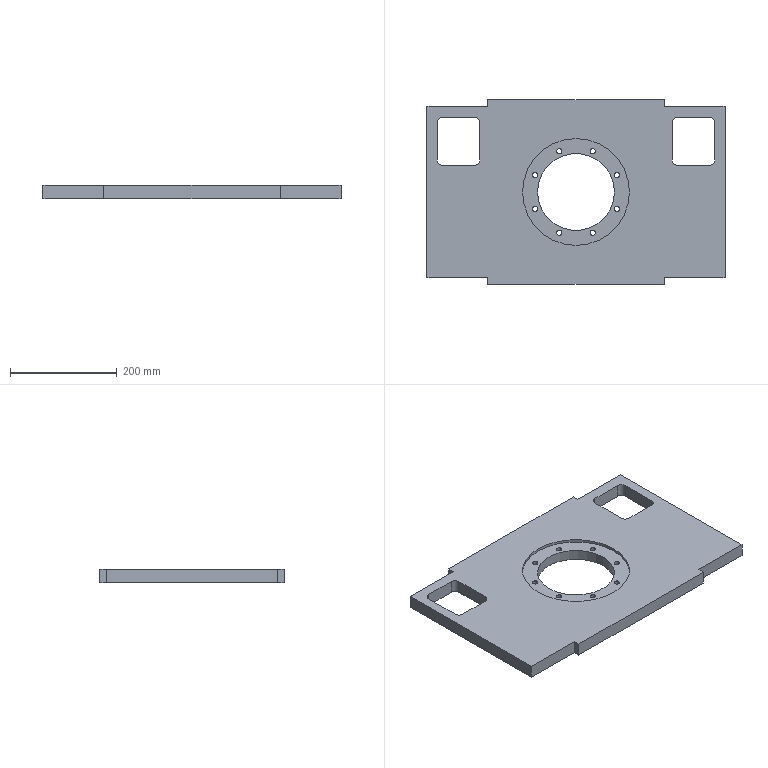Component | NX | CH3404_5-6 | 1 solid | 57 faces | volume 3826086 mm3 | plane 23 | cylinder 18 | cone 16 | commonest cylinder face diameters 9.5 x8 20 x8 144 x1 200 x1